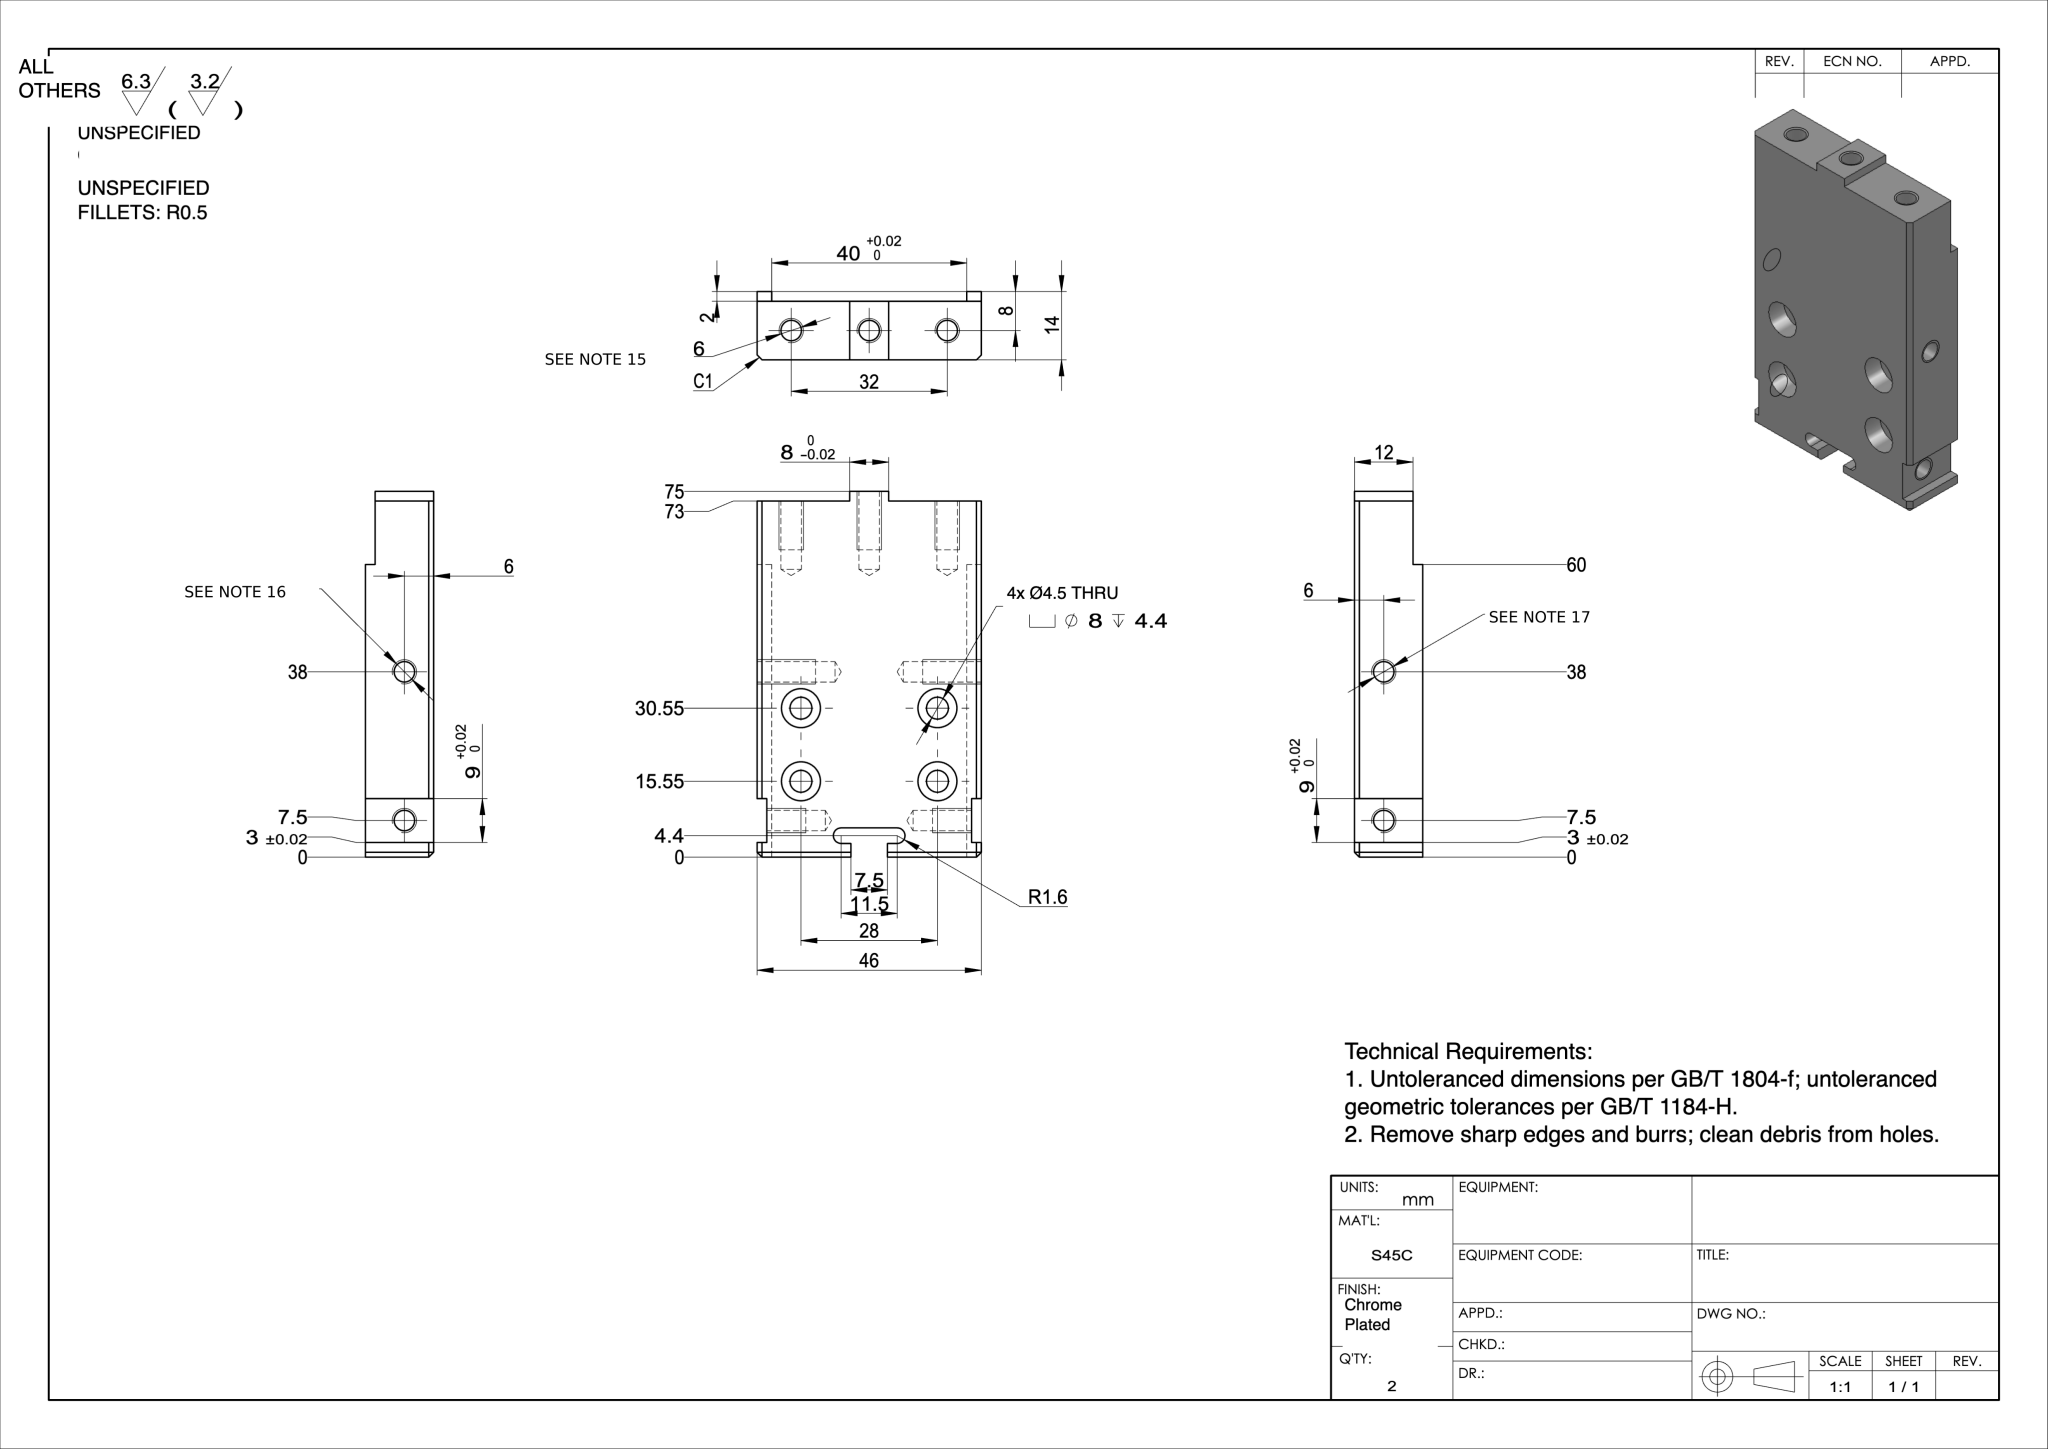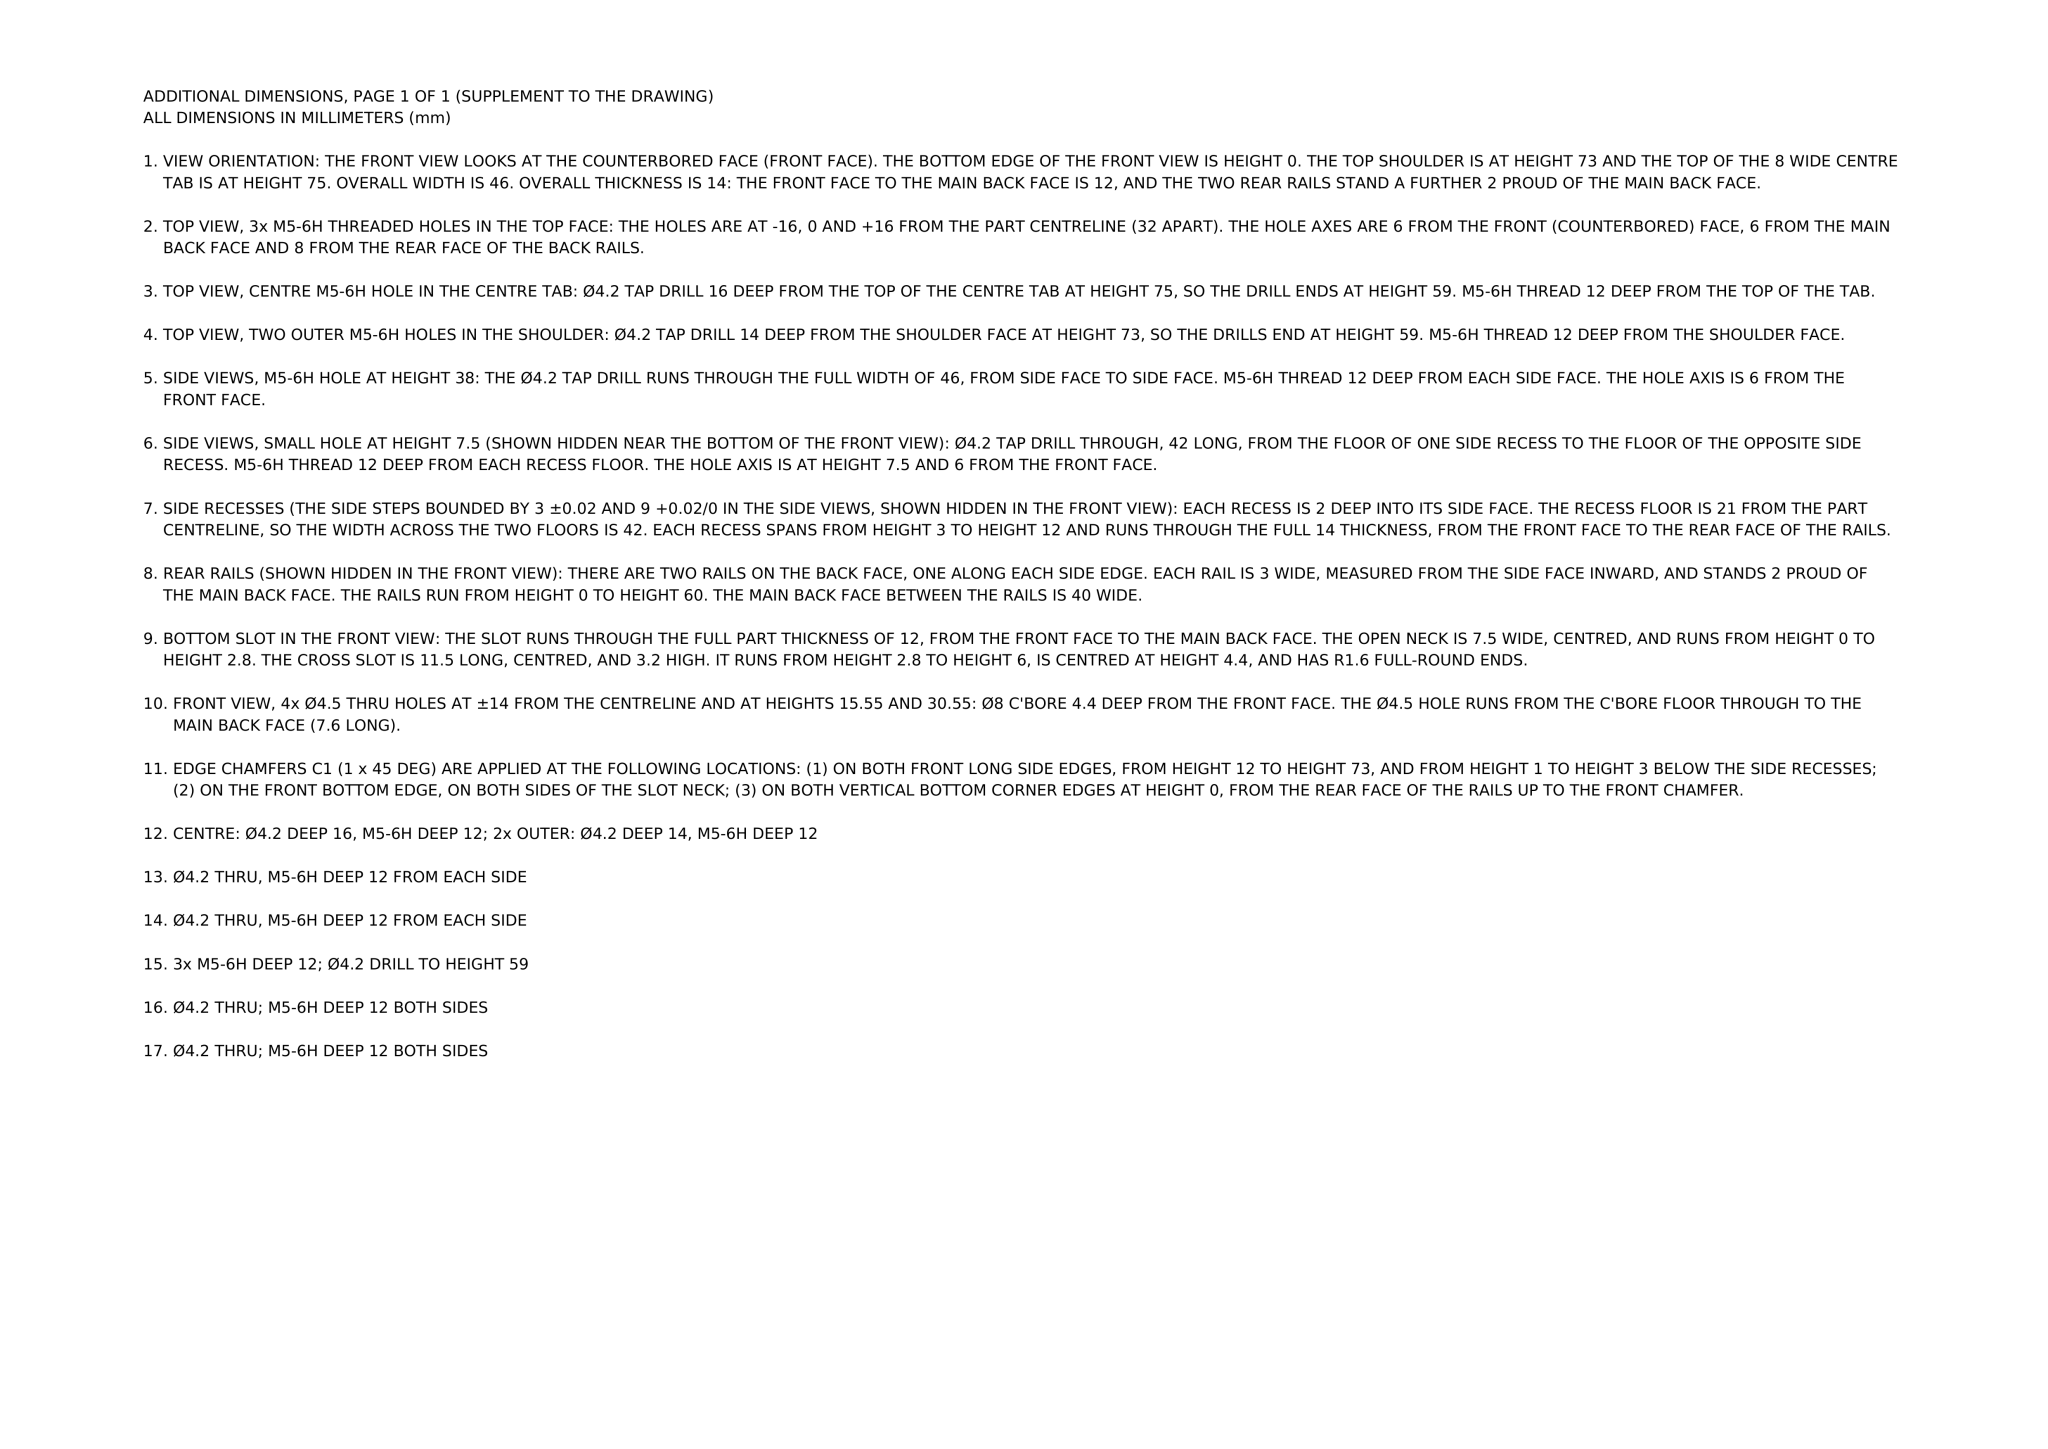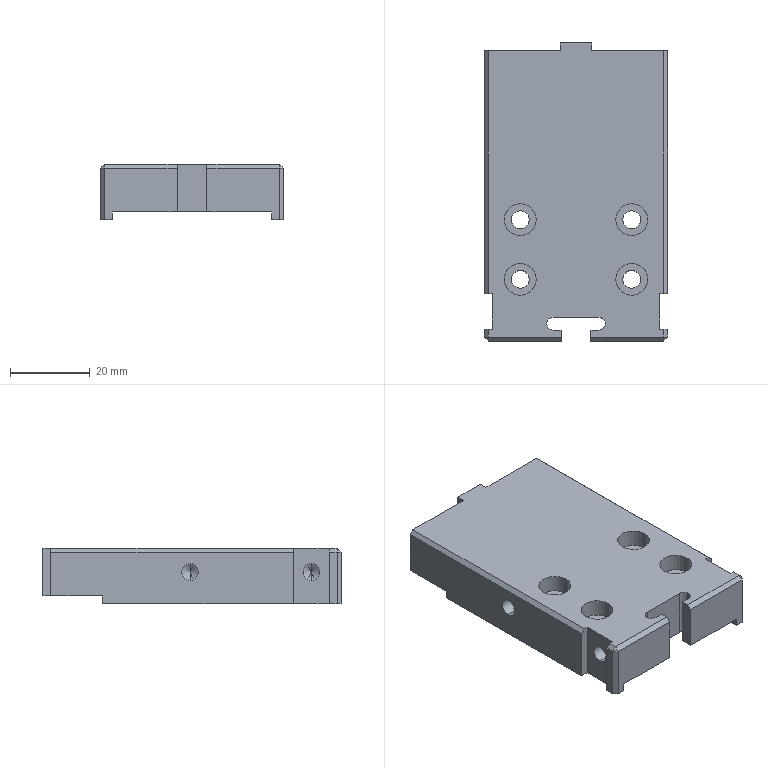Part | NX | mm | 1 solid | 91 faces | box 46 x 75 x 14 mm | volume 37024 mm3 | plane 44 | cylinder 33 | cone 14 | commonest cylinder face diameters 4.2 x14 8 x8 4.5 x8 3.2 x3